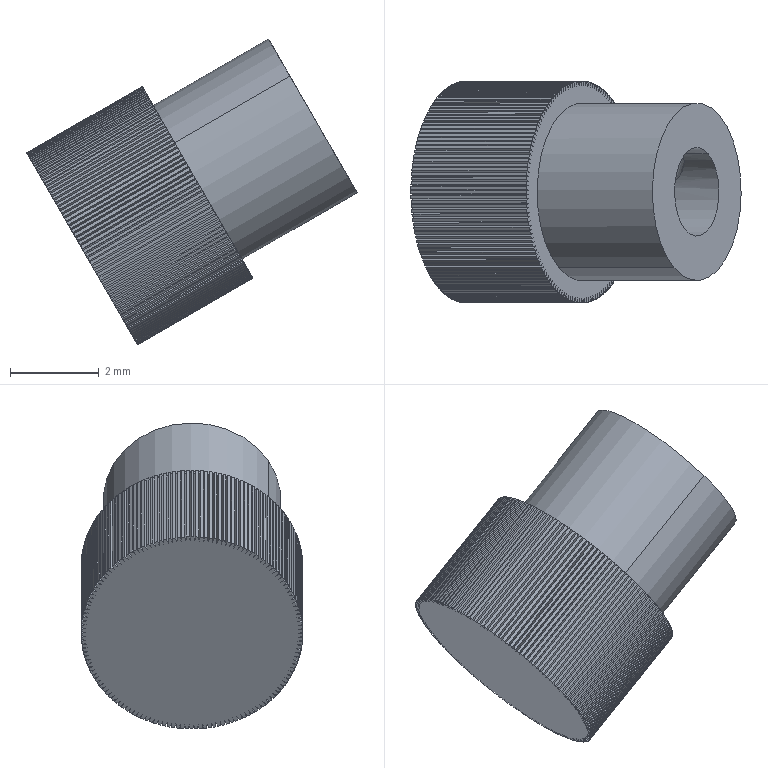Component | SolidWorks | SliderNut1-1 | 1 solid | 460 faces | volume 86 mm3 | plane 304 | cylinder 156 | commonest cylinder face diameters 5 x150 1.6 x2 2 x2 4 x2